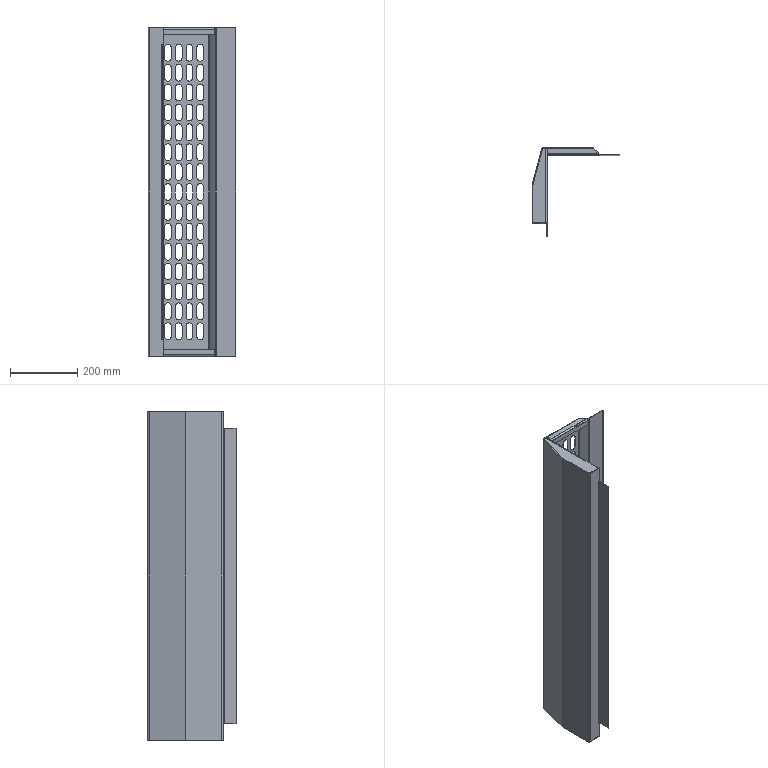Component | NX | UPPER_BEAM_FRONT | 5 solids | 332 faces | volume 1038660 mm3 | plane 182 | cylinder 148 | spline 2 | commonest cylinder face diameters 20 x120 10 x10 6 x10 7 x8